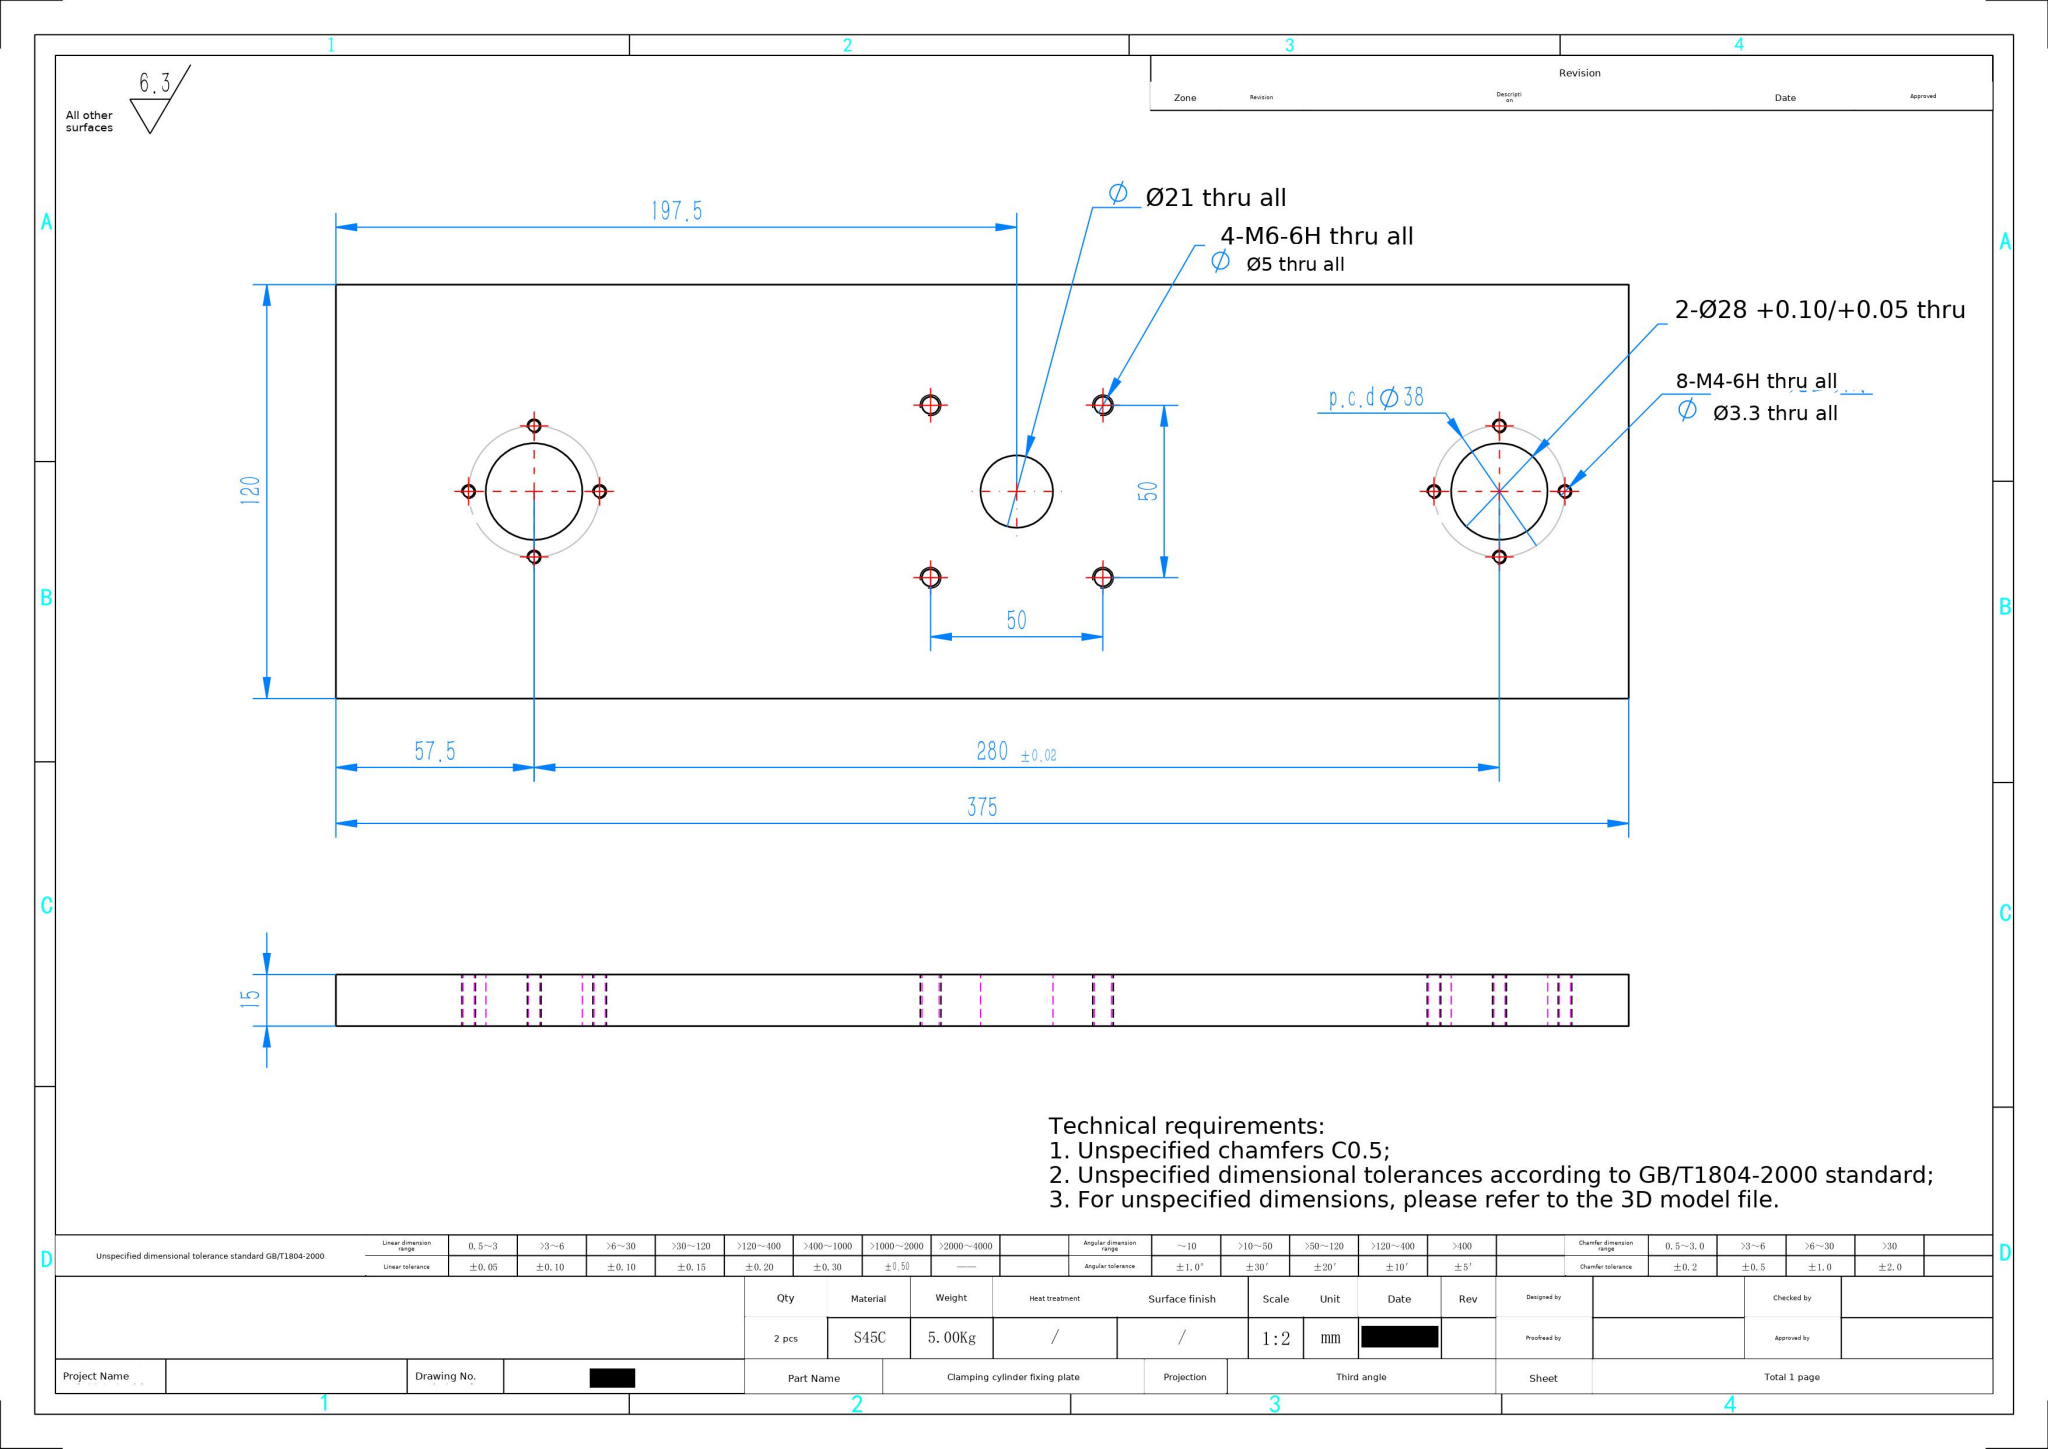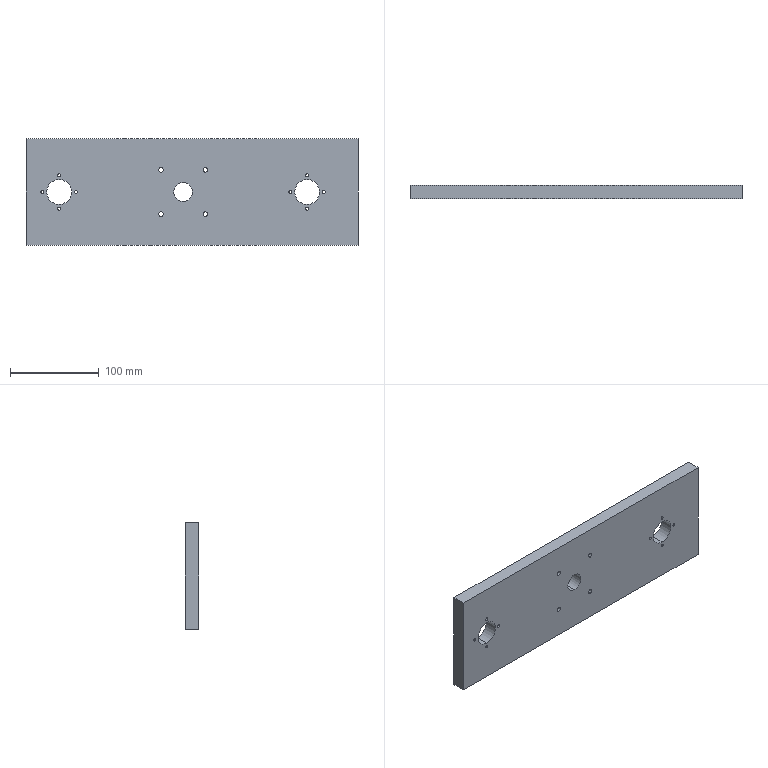Part | SolidWorks | mm | material S45C | 1 solid | 36 faces | box 375 x 15 x 120 mm | volume 649128 mm3 | cylinder 30 | plane 6 | commonest cylinder face diameters 3.3 x16 5 x8 28 x4 21 x2
build123d program:
from build123d import *

# Parameters (mm, degrees)
SKETCH1_W                  = 375
SKETCH1_H                  = 120
BOSS_EXTRUDE1_DEPTH        = 15
SKETCH2_R                  = 14
CUT_EXTRUDE1_DEPTH         = 198.437
F_21_0_21_DIAMETER_HOLE1_D = 21
M6_TAPPED_HOLE1_D          = 5
M4_TAPPED_HOLE1_D          = 3.3


with BuildPart() as part:
    # Sketch1 → Boss-Extrude1 (new body)
    with BuildSketch(Plane(origin=(0, 0, 0), x_dir=(1, 0, 0), z_dir=(0, 1, 0))):
        Rectangle(SKETCH1_W, SKETCH1_H)
    extrude(amount=BOSS_EXTRUDE1_DEPTH)

    # Sketch2 → Cut-Extrude1 (cut, through all)
    with BuildSketch(Plane.XZ):
        with Locations(Location((-150, 0, 0), (0, 0, 270))):
            Circle(SKETCH2_R)
        with Locations(Location((130, 0, 0), (0, 0, 90))):
            Circle(SKETCH2_R)
    extrude(amount=-CUT_EXTRUDE1_DEPTH, mode=Mode.SUBTRACT)

    # 21.0 _21_ Diameter Hole1 (through all)
    with Locations(Plane(origin=(0, 15, 0), x_dir=(1, 0, 0), z_dir=(0, 1, 0))):
        with Locations((-10, 0)):
            Hole(F_21_0_21_DIAMETER_HOLE1_D / 2)

    # M6 Tapped Hole1 (through all)
    with Locations(Plane(origin=(0, 15, 0), x_dir=(1, 0, 0), z_dir=(0, 1, 0))):
        with Locations((15, -25), (-35, 25), (15, 25), (-35, -25)):
            Hole(M6_TAPPED_HOLE1_D / 2)

    # M4 Tapped Hole1 (through all)
    with Locations(Plane(origin=(0, 0, 0), x_dir=(-1, 0, 0), z_dir=(0, -1, 0))):
        with Locations((-111, 0), (-149, 0), (-130, -19), (-130, 19), (169, 0), (131, 0), (150, -19), (150, 19)):
            Hole(M4_TAPPED_HOLE1_D / 2)


solid = part.part